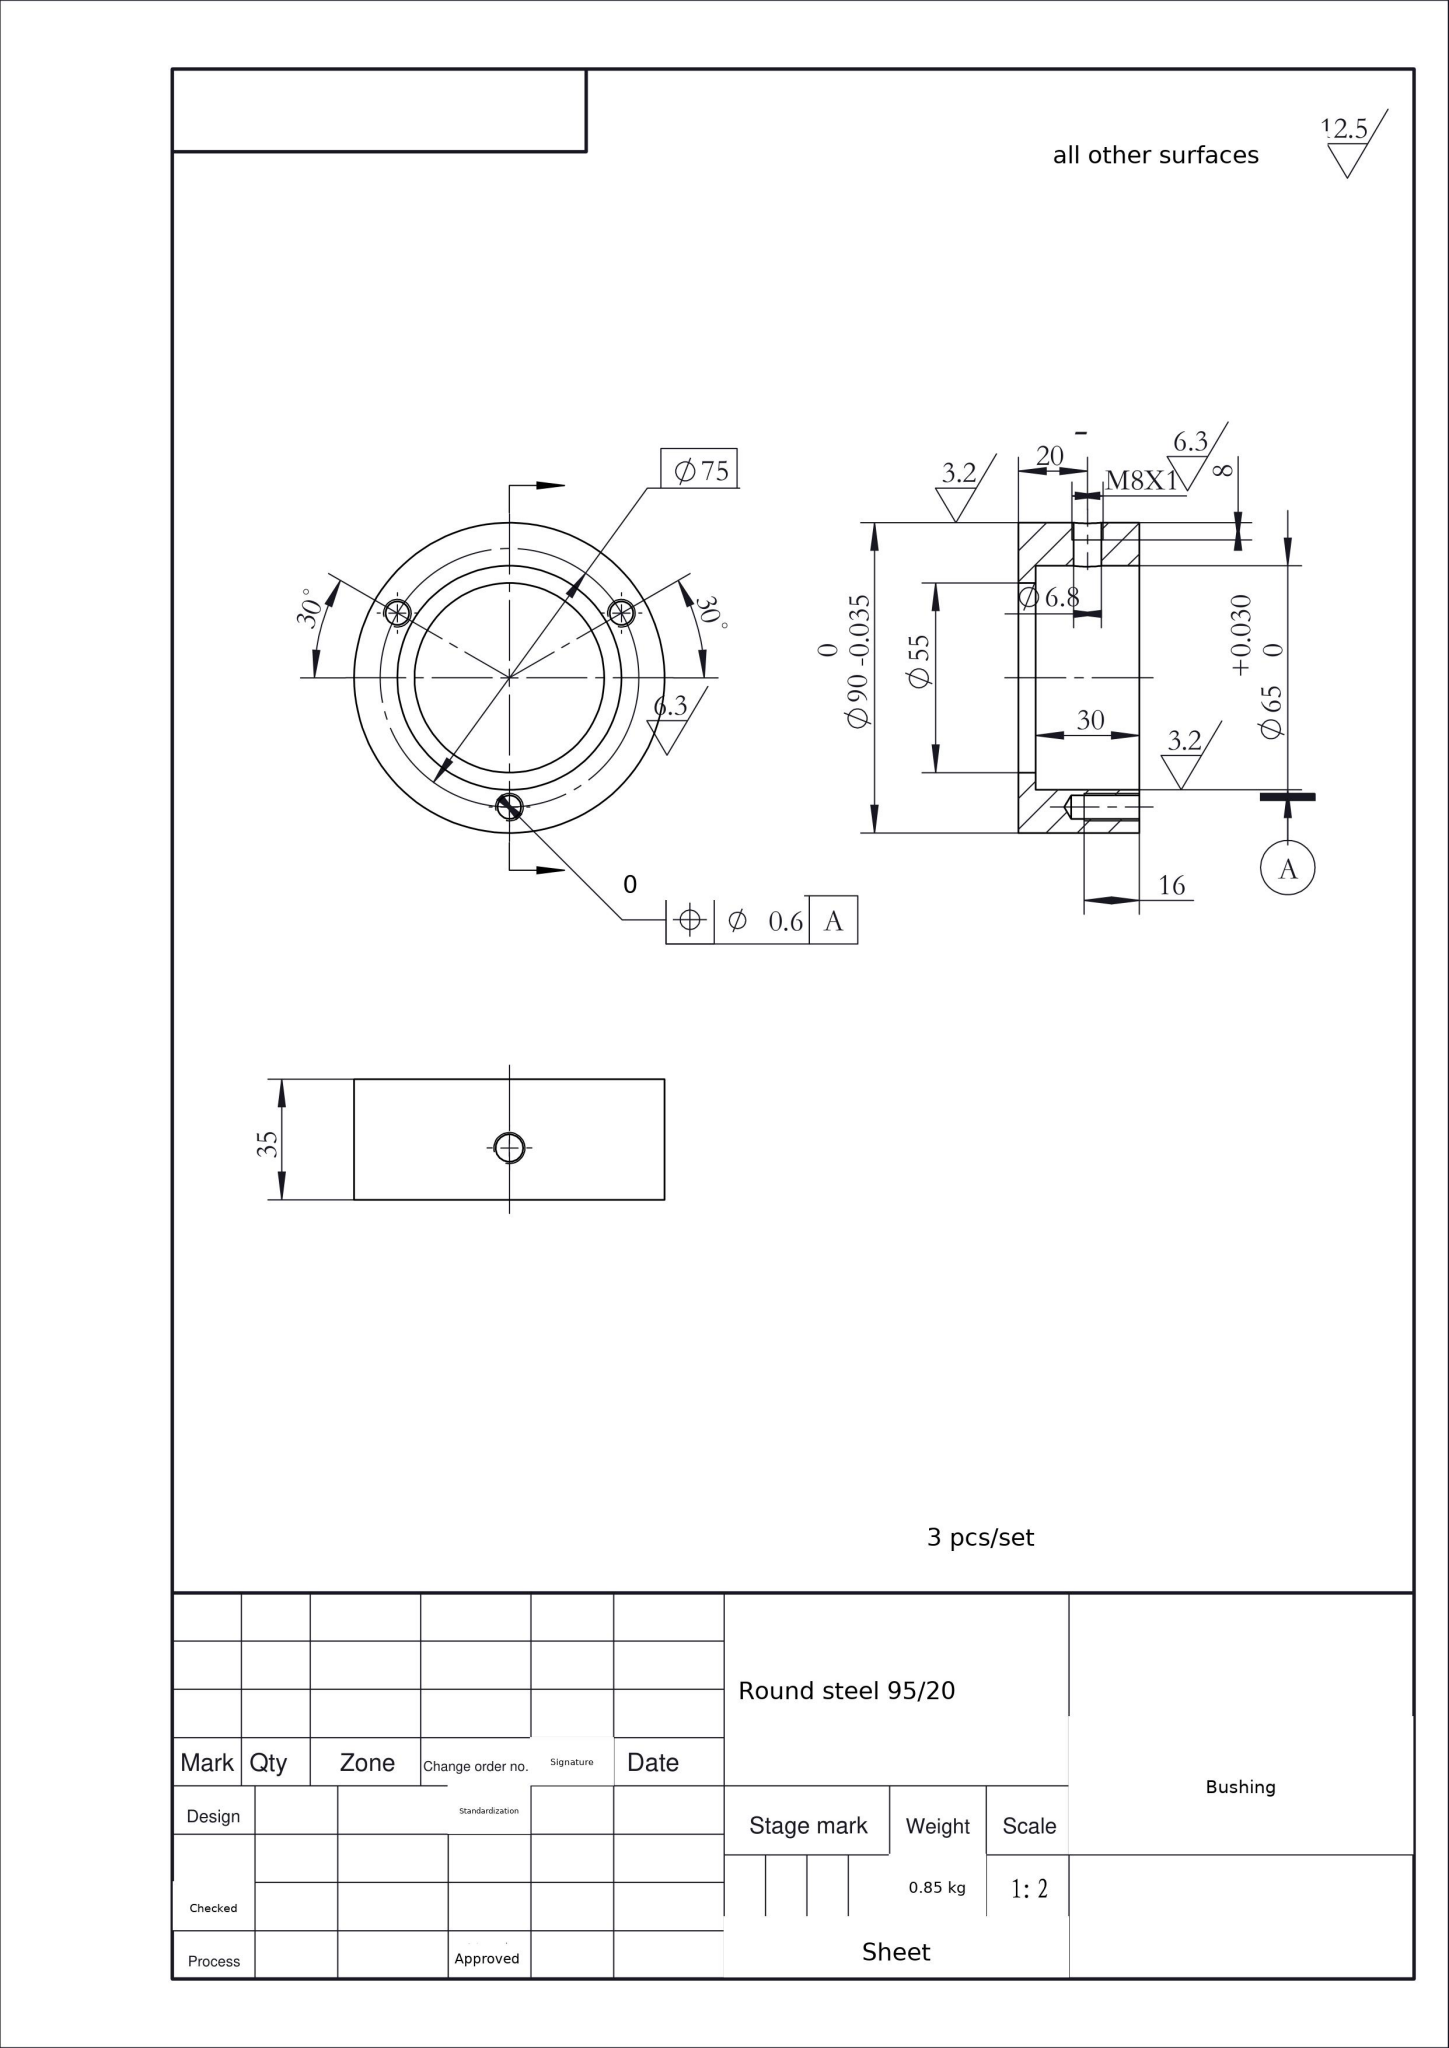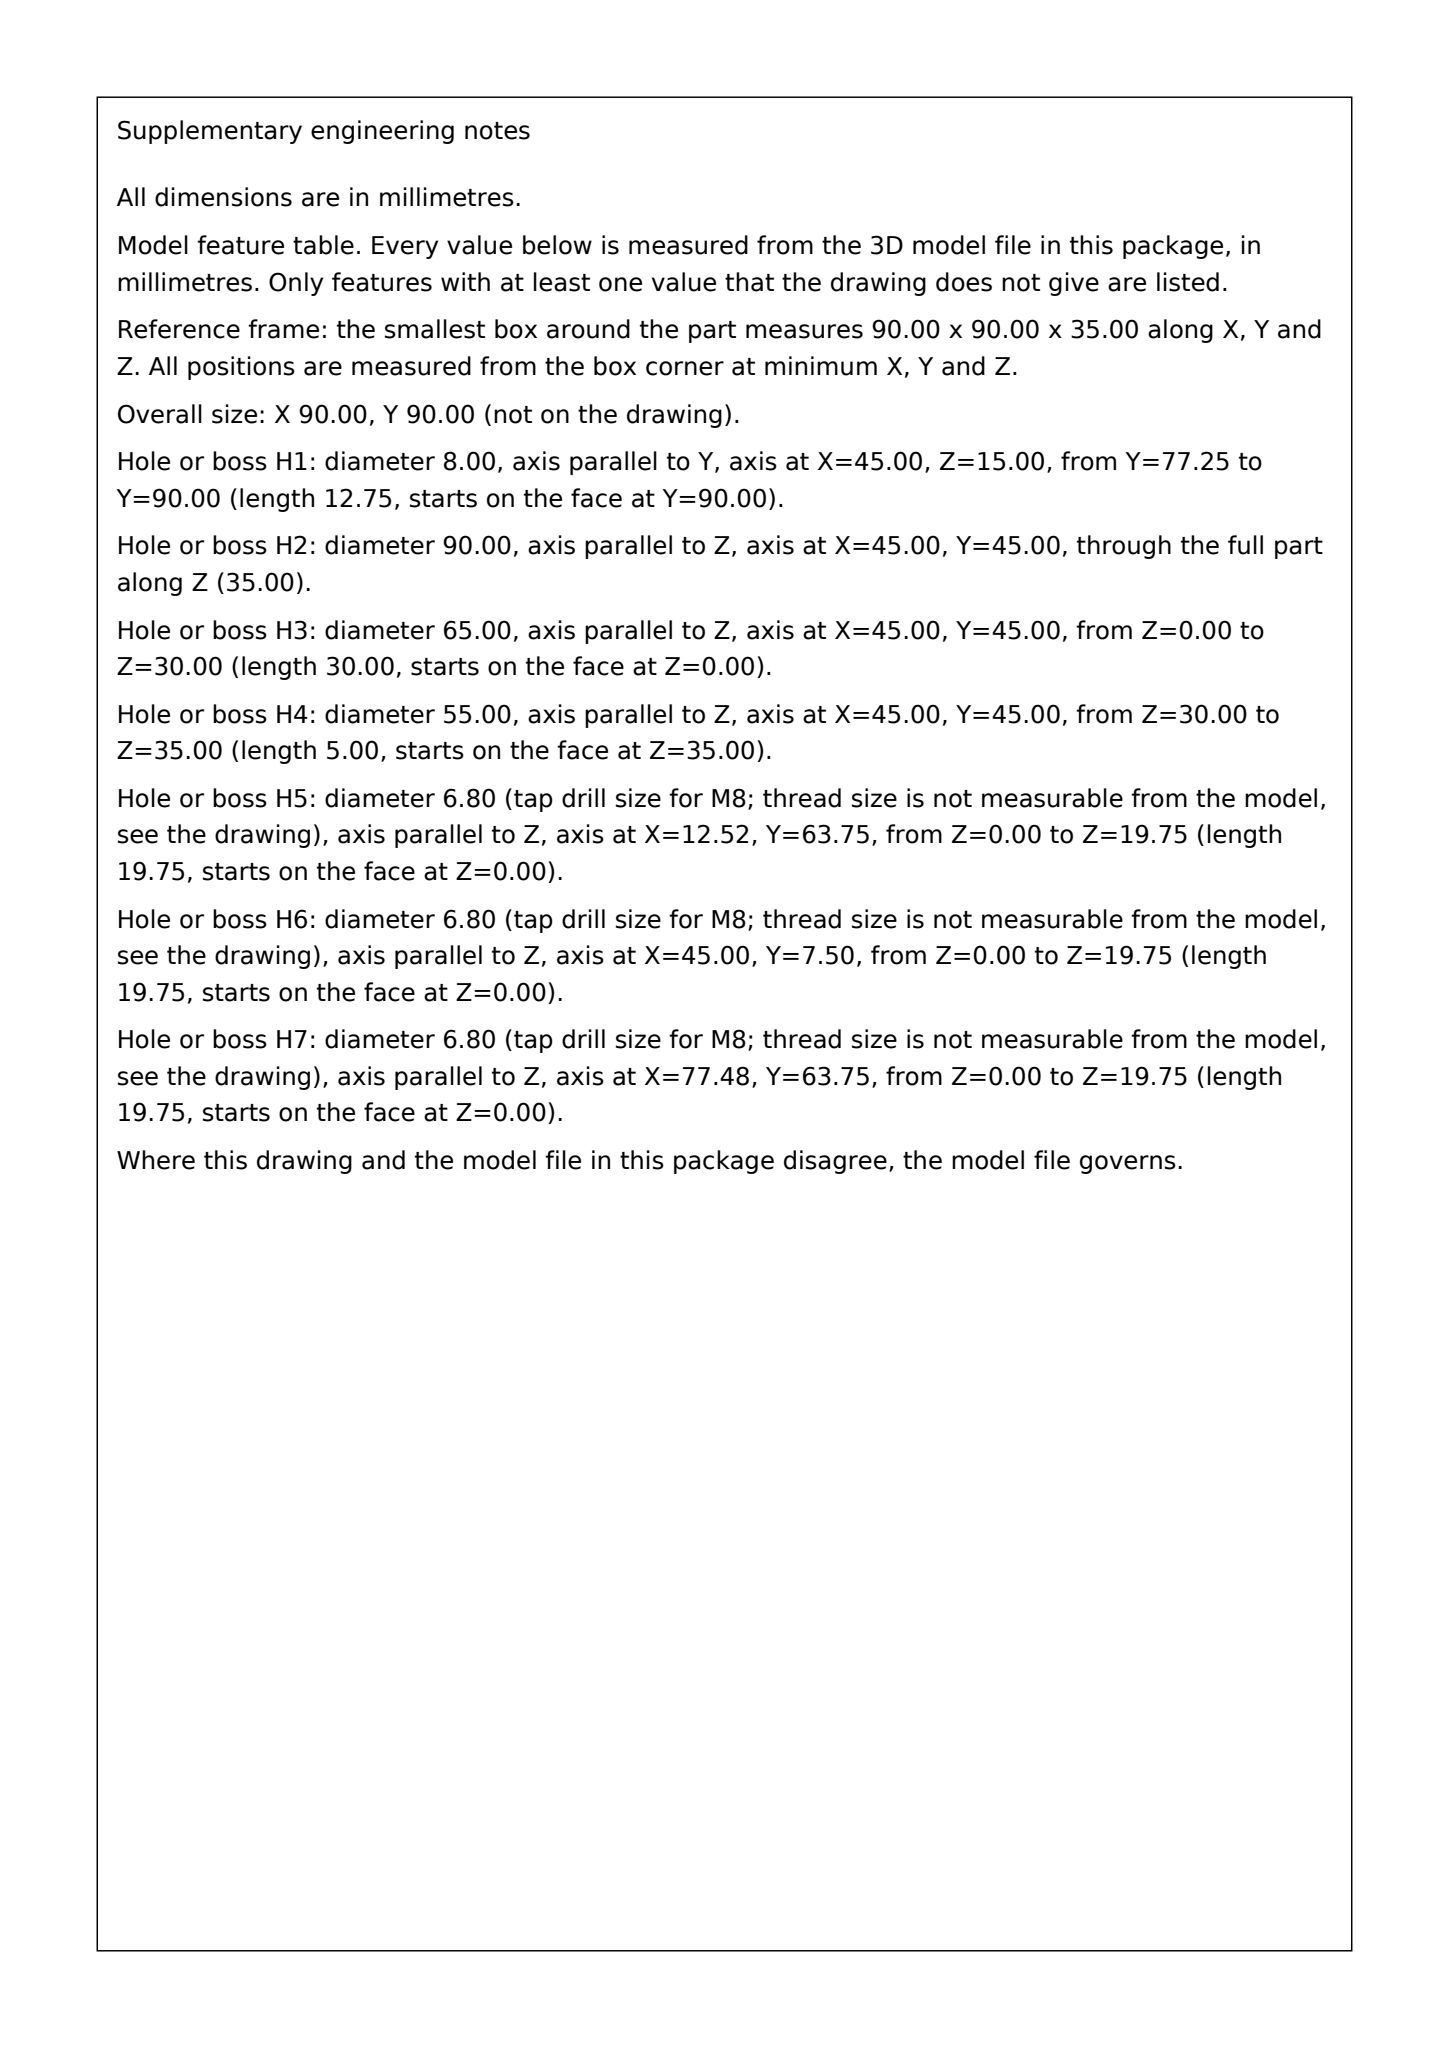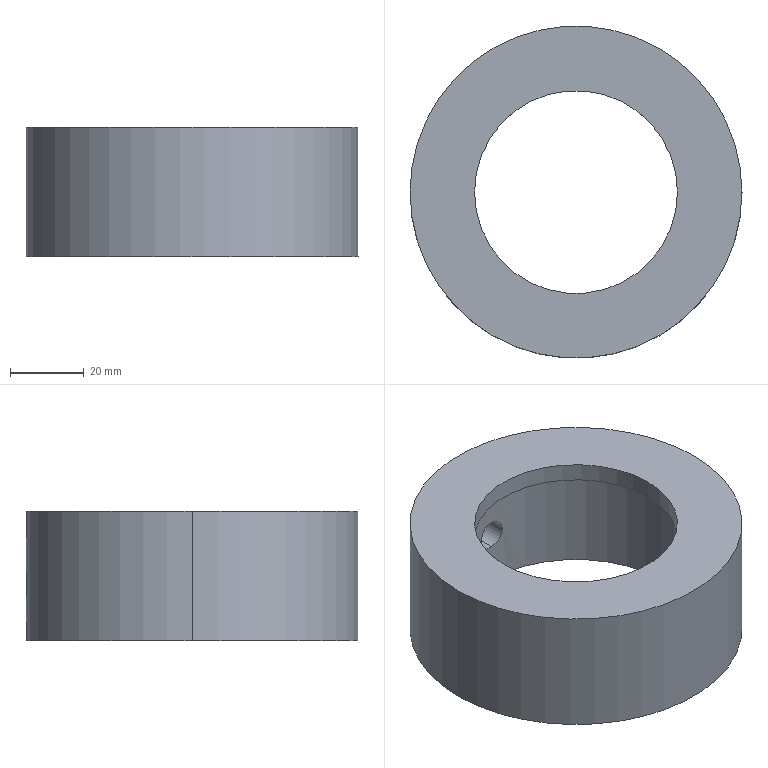Part | SolidWorks | mm | material Round steel 95/20 | 1 solid | 23 faces | box 90 x 90 x 35 mm | volume 108376 mm3 | cylinder 14 | cone 6 | plane 3 | commonest cylinder face diameters 6.8 x6 8 x2 65 x2 55 x2 90 x2
build123d program:
from build123d import *

# Parameters (mm, degrees)
SKETCH1_R               = 45
BOSS_EXTRUDE1_DEPTH     = 35
SKETCH2_R               = 27.5
CUT_EXTRUDE1_DEPTH      = 5
SKETCH3_R               = 32.5
CUT_EXTRUDE2_DEPTH      = 30
M8_TAPPED_HOLE1_D       = 6.8
M8_TAPPED_HOLE1_DEPTH   = 19.75
M8_TAPPED_HOLE1_TIP     = 2.043
CUT_EXTRUDE3_REACH      = 108.536
CUT_EXTRUDE3_END_RADIUS = 32.5
SKETCH9_R               = 4


with BuildPart() as part:
    # Sketch1 → Boss-Extrude1 (new body)
    with BuildSketch(Plane.XY):
        Circle(SKETCH1_R)
    extrude(amount=BOSS_EXTRUDE1_DEPTH)

    # Sketch2 → Cut-Extrude1 (cut)
    with BuildSketch(Plane.XY.offset(35)):
        Circle(SKETCH2_R)
    extrude(amount=-CUT_EXTRUDE1_DEPTH, mode=Mode.SUBTRACT)

    # Sketch3 → Cut-Extrude2 (cut)
    with BuildSketch(Plane(origin=(0, 0, 0), x_dir=(-1, 0, 0), z_dir=(0, 0, -1))):
        Circle(SKETCH3_R)
    extrude(amount=-CUT_EXTRUDE2_DEPTH, mode=Mode.SUBTRACT)

    # M8 Tapped Hole1
    with Locations(Plane(origin=(32.476, 18.75, 0), x_dir=(-1, 0, 0), z_dir=(0, 0, -1))):
        with Locations((0, 0), (64.952, 0), (32.476, -56.25)):
            Hole(M8_TAPPED_HOLE1_D / 2, depth=M8_TAPPED_HOLE1_DEPTH)
            with Locations((0, 0, -(M8_TAPPED_HOLE1_DEPTH + M8_TAPPED_HOLE1_TIP / 2))):  # 118° drill point
                Cone(0, M8_TAPPED_HOLE1_D / 2, M8_TAPPED_HOLE1_TIP, mode=Mode.SUBTRACT)

    # Cut-Extrude3: up to this cylinder (the profile starts outside it)
    cut_extrude3_end = Plane(origin=(0, 0, 15), z_dir=(0, 0, -1)) * Cylinder(CUT_EXTRUDE3_END_RADIUS, 283.072, mode=Mode.PRIVATE)
    # Sketch9 → Cut-Extrude3 (cut, up to the surface)
    with BuildSketch(Plane(origin=(0, 45, 0), x_dir=(1, 0, 0), z_dir=(0, 1, 0)), mode=Mode.PRIVATE) as cut_extrude3_sk1:
        with Locations(Location((0, -15, 0), (0, 0, 270))):
            Circle(SKETCH9_R)
    cut_extrude3_tool1 = extrude(cut_extrude3_sk1.sketch, amount=-CUT_EXTRUDE3_REACH, mode=Mode.PRIVATE) - cut_extrude3_end
    add(cut_extrude3_tool1.solids().sort_by_distance((0, 45, 15))[0], mode=Mode.SUBTRACT)


solid = part.part
STEP:
#1=CARTESIAN_POINT('',(0.,32.5,19.));
#2=VERTEX_POINT('',#1);
#3=CARTESIAN_POINT('',(-0.,32.5,11.));
#4=VERTEX_POINT('',#3);
#5=CARTESIAN_POINT('',(0.,32.5,19.));
#6=CARTESIAN_POINT('',(-0.2646,32.5,19.));
#7=CARTESIAN_POINT('',(-0.5246,32.497,18.974));
#8=CARTESIAN_POINT('',(-1.036,32.484,18.872));
#9=CARTESIAN_POINT('',(-1.29,32.475,18.795));
#10=CARTESIAN_POINT('',(-1.775,32.452,18.594));
#11=CARTESIAN_POINT('',(-2.004,32.439,18.471));
#12=CARTESIAN_POINT('',(-2.439,32.409,18.181));
#13=CARTESIAN_POINT('',(-2.645,32.393,18.012));
#14=CARTESIAN_POINT('',(-3.013,32.361,17.643));
#15=CARTESIAN_POINT('',(-3.179,32.345,17.442));
#16=CARTESIAN_POINT('',(-3.471,32.314,17.005));
#17=CARTESIAN_POINT('',(-3.595,32.301,16.773));
#18=CARTESIAN_POINT('',(-3.795,32.278,16.291));
#19=CARTESIAN_POINT('',(-3.872,32.269,16.039));
#20=CARTESIAN_POINT('',(-3.974,32.256,15.522));
#21=CARTESIAN_POINT('',(-4.,32.253,15.263));
#22=CARTESIAN_POINT('',(-4.,32.253,14.74));
#23=CARTESIAN_POINT('',(-3.974,32.256,14.475));
#24=CARTESIAN_POINT('',(-3.872,32.269,13.962));
#25=CARTESIAN_POINT('',(-3.796,32.278,13.712));
#26=CARTESIAN_POINT('',(-3.596,32.301,13.228));
#27=CARTESIAN_POINT('',(-3.47,32.315,12.994));
#28=CARTESIAN_POINT('',(-3.181,32.344,12.561));
#29=CARTESIAN_POINT('',(-3.015,32.36,12.359));
#30=CARTESIAN_POINT('',(-2.642,32.393,11.985));
#31=CARTESIAN_POINT('',(-2.44,32.409,11.82));
#32=CARTESIAN_POINT('',(-2.007,32.439,11.53));
#33=CARTESIAN_POINT('',(-1.773,32.452,11.405));
#34=CARTESIAN_POINT('',(-1.289,32.475,11.204));
#35=CARTESIAN_POINT('',(-1.04,32.484,11.129));
#36=CARTESIAN_POINT('',(-0.5265,32.497,11.026));
#37=CARTESIAN_POINT('',(-0.2612,32.5,11.));
#38=CARTESIAN_POINT('',(-0.,32.5,11.));
#39=B_SPLINE_CURVE_WITH_KNOTS('',3,(#5,#6,#7,#8,#9,#10,#11,#12,#13,#14,#15,#16,#17,#18,#19,#20,#21,#22,#23,#24,#25,#26,#27,#28,#29,#30,#31,#32,#33,#34,#35,#36,#37,#38),.UNSPECIFIED.,.F.,.F.,(4,2,2,2,2,2,2,2,2,2,2,2,2,2,2,2,4),(0.,0.0007824,0.001565,0.002347,0.003129,0.003912,0.004694,0.005476,0.006259,0.007041,0.007824,0.008606,0.009388,0.01017,0.01095,0.01174,0.01252),.UNSPECIFIED.);
#40=EDGE_CURVE('',#2,#4,#39,.T.);
#41=ORIENTED_EDGE('',*,*,#40,.T.);
#42=CARTESIAN_POINT('',(-0.,45.,11.));
#43=VERTEX_POINT('',#42);
#44=CARTESIAN_POINT('',(-0.,-45.001,11.));
#45=DIRECTION('',(-0.,1.,-0.));
#46=VECTOR('',#45,1000.);
#47=LINE('',#44,#46);
#48=EDGE_CURVE('',#4,#43,#47,.T.);
#49=ORIENTED_EDGE('',*,*,#48,.T.);
#50=CARTESIAN_POINT('',(-0.,45.,19.));
#51=VERTEX_POINT('',#50);
#52=CARTESIAN_POINT('',(-0.,45.,11.));
#53=CARTESIAN_POINT('',(-0.2611,45.,11.));
#54=CARTESIAN_POINT('',(-0.5206,44.998,11.025));
#55=CARTESIAN_POINT('',(-1.037,44.989,11.128));
#56=CARTESIAN_POINT('',(-1.289,44.982,11.205));
#57=CARTESIAN_POINT('',(-1.771,44.966,11.404));
#58=CARTESIAN_POINT('',(-2.003,44.956,11.528));
#59=CARTESIAN_POINT('',(-2.441,44.934,11.82));
#60=CARTESIAN_POINT('',(-2.642,44.923,11.985));
#61=CARTESIAN_POINT('',(-3.011,44.9,12.354));
#62=CARTESIAN_POINT('',(-3.18,44.888,12.559));
#63=CARTESIAN_POINT('',(-3.47,44.866,12.994));
#64=CARTESIAN_POINT('',(-3.593,44.856,13.224));
#65=CARTESIAN_POINT('',(-3.794,44.84,13.707));
#66=CARTESIAN_POINT('',(-3.872,44.833,13.962));
#67=CARTESIAN_POINT('',(-3.974,44.824,14.473));
#68=CARTESIAN_POINT('',(-4.,44.822,14.733));
#69=CARTESIAN_POINT('',(-4.,44.822,15.261));
#70=CARTESIAN_POINT('',(-3.974,44.824,15.522));
#71=CARTESIAN_POINT('',(-3.873,44.833,16.033));
#72=CARTESIAN_POINT('',(-3.796,44.84,16.287));
#73=CARTESIAN_POINT('',(-3.596,44.856,16.771));
#74=CARTESIAN_POINT('',(-3.473,44.866,17.001));
#75=CARTESIAN_POINT('',(-3.183,44.887,17.436));
#76=CARTESIAN_POINT('',(-3.015,44.899,17.642));
#77=CARTESIAN_POINT('',(-2.646,44.923,18.011));
#78=CARTESIAN_POINT('',(-2.445,44.934,18.177));
#79=CARTESIAN_POINT('',(-2.008,44.956,18.469));
#80=CARTESIAN_POINT('',(-1.776,44.966,18.594));
#81=CARTESIAN_POINT('',(-1.295,44.982,18.794));
#82=CARTESIAN_POINT('',(-1.043,44.989,18.871));
#83=CARTESIAN_POINT('',(-0.5259,44.998,18.974));
#84=CARTESIAN_POINT('',(-0.2644,45.,19.));
#85=CARTESIAN_POINT('',(-0.,45.,19.));
#86=B_SPLINE_CURVE_WITH_KNOTS('',3,(#52,#53,#54,#55,#56,#57,#58,#59,#60,#61,#62,#63,#64,#65,#66,#67,#68,#69,#70,#71,#72,#73,#74,#75,#76,#77,#78,#79,#80,#81,#82,#83,#84,#85),.UNSPECIFIED.,.F.,.F.,(4,2,2,2,2,2,2,2,2,2,2,2,2,2,2,2,4),(0.01251,0.01329,0.01408,0.01486,0.01564,0.01642,0.0172,0.01798,0.01877,0.01955,0.02033,0.02111,0.02189,0.02268,0.02346,0.02424,0.02502),.UNSPECIFIED.);
#87=EDGE_CURVE('',#43,#51,#86,.T.);
#88=ORIENTED_EDGE('',*,*,#87,.T.);
#89=CARTESIAN_POINT('',(-0.,-45.001,19.));
#90=DIRECTION('',(-0.,1.,-0.));
#91=VECTOR('',#90,1000.);
#92=LINE('',#89,#91);
#93=EDGE_CURVE('',#2,#51,#92,.T.);
#94=ORIENTED_EDGE('',*,*,#93,.F.);
#95=EDGE_LOOP('',(#41,#49,#88,#94));
#96=FACE_OUTER_BOUND('',#95,.T.);
#97=CARTESIAN_POINT('',(-0.,-45.001,15.));
#98=DIRECTION('',(-0.,1.,-0.));
#99=DIRECTION('',(-0.,0.,1.));
#100=AXIS2_PLACEMENT_3D('',#97,#98,#99);
#101=CYLINDRICAL_SURFACE('',#100,4.);
#102=ADVANCED_FACE('',(#96),#101,.F.);
#103=CARTESIAN_POINT('',(35.876,18.75,19.75));
#104=VERTEX_POINT('',#103);
#105=CARTESIAN_POINT('',(29.076,18.75,19.75));
#106=VERTEX_POINT('',#105);
#107=CARTESIAN_POINT('',(32.476,18.75,19.75));
#108=DIRECTION('',(0.,0.,-1.));
#109=DIRECTION('',(-1.,0.,0.));
#110=AXIS2_PLACEMENT_3D('',#107,#108,#109);
#111=CIRCLE('',#110,3.4);
#112=EDGE_CURVE('',#104,#106,#111,.T.);
#113=ORIENTED_EDGE('',*,*,#112,.F.);
#114=CARTESIAN_POINT('',(35.876,18.75,-0.));
#115=VERTEX_POINT('',#114);
#116=CARTESIAN_POINT('',(35.876,18.75,-0.));
#117=DIRECTION('',(0.,0.,-1.));
#118=VECTOR('',#117,1000.);
#119=LINE('',#116,#118);
#120=EDGE_CURVE('',#104,#115,#119,.T.);
#121=ORIENTED_EDGE('',*,*,#120,.T.);
#122=CARTESIAN_POINT('',(29.076,18.75,-0.));
#123=VERTEX_POINT('',#122);
#124=CARTESIAN_POINT('',(32.476,18.75,-0.));
#125=DIRECTION('',(0.,0.,-1.));
#126=DIRECTION('',(-1.,0.,0.));
#127=AXIS2_PLACEMENT_3D('',#124,#125,#126);
#128=CIRCLE('',#127,3.4);
#129=EDGE_CURVE('',#115,#123,#128,.T.);
#130=ORIENTED_EDGE('',*,*,#129,.T.);
#131=CARTESIAN_POINT('',(29.076,18.75,-0.));
#132=DIRECTION('',(0.,0.,-1.));
#133=VECTOR('',#132,1000.);
#134=LINE('',#131,#133);
#135=EDGE_CURVE('',#106,#123,#134,.T.);
#136=ORIENTED_EDGE('',*,*,#135,.F.);
#137=EDGE_LOOP('',(#113,#121,#130,#136));
#138=FACE_OUTER_BOUND('',#137,.T.);
#139=CARTESIAN_POINT('',(32.476,18.75,-0.));
#140=DIRECTION('',(0.,0.,-1.));
#141=DIRECTION('',(-1.,0.,0.));
#142=AXIS2_PLACEMENT_3D('',#139,#140,#141);
#143=CYLINDRICAL_SURFACE('',#142,3.4);
#144=ADVANCED_FACE('',(#138),#143,.F.);
#145=CARTESIAN_POINT('',(32.476,18.75,21.793));
#146=VERTEX_POINT('',#145);
#147=CARTESIAN_POINT('',(29.076,18.75,19.75));
#148=DIRECTION('',(-0.8572,0.,-0.515));
#149=VECTOR('',#148,1000.);
#150=LINE('',#147,#149);
#151=EDGE_CURVE('',#146,#106,#150,.T.);
#152=ORIENTED_EDGE('',*,*,#151,.F.);
#153=CARTESIAN_POINT('',(35.876,18.75,19.75));
#154=DIRECTION('',(0.8572,-0.,-0.515));
#155=VECTOR('',#154,1000.);
#156=LINE('',#153,#155);
#157=EDGE_CURVE('',#146,#104,#156,.T.);
#158=ORIENTED_EDGE('',*,*,#157,.T.);
#159=ORIENTED_EDGE('',*,*,#112,.T.);
#160=EDGE_LOOP('',(#152,#158,#159));
#161=FACE_OUTER_BOUND('',#160,.T.);
#162=CARTESIAN_POINT('',(32.476,18.75,19.75));
#163=DIRECTION('',(0.,0.,-1.));
#164=DIRECTION('',(-1.,0.,0.));
#165=AXIS2_PLACEMENT_3D('',#162,#163,#164);
#166=CONICAL_SURFACE('',#165,3.4,1.03);
#167=ADVANCED_FACE('',(#161),#166,.F.);
#168=CARTESIAN_POINT('',(-29.076,18.75,19.75));
#169=VERTEX_POINT('',#168);
#170=CARTESIAN_POINT('',(-35.876,18.75,19.75));
#171=VERTEX_POINT('',#170);
#172=CARTESIAN_POINT('',(-32.476,18.75,19.75));
#173=DIRECTION('',(0.,0.,-1.));
#174=DIRECTION('',(-1.,0.,0.));
#175=AXIS2_PLACEMENT_3D('',#172,#173,#174);
#176=CIRCLE('',#175,3.4);
#177=EDGE_CURVE('',#169,#171,#176,.T.);
#178=ORIENTED_EDGE('',*,*,#177,.F.);
#179=CARTESIAN_POINT('',(-29.076,18.75,-0.));
#180=VERTEX_POINT('',#179);
#181=CARTESIAN_POINT('',(-29.076,18.75,-0.));
#182=DIRECTION('',(0.,0.,-1.));
#183=VECTOR('',#182,1000.);
#184=LINE('',#181,#183);
#185=EDGE_CURVE('',#169,#180,#184,.T.);
#186=ORIENTED_EDGE('',*,*,#185,.T.);
#187=CARTESIAN_POINT('',(-35.876,18.75,-0.));
#188=VERTEX_POINT('',#187);
#189=CARTESIAN_POINT('',(-32.476,18.75,-0.));
#190=DIRECTION('',(0.,0.,-1.));
#191=DIRECTION('',(-1.,0.,0.));
#192=AXIS2_PLACEMENT_3D('',#189,#190,#191);
#193=CIRCLE('',#192,3.4);
#194=EDGE_CURVE('',#180,#188,#193,.T.);
#195=ORIENTED_EDGE('',*,*,#194,.T.);
#196=CARTESIAN_POINT('',(-35.876,18.75,-0.));
#197=DIRECTION('',(0.,0.,-1.));
#198=VECTOR('',#197,1000.);
#199=LINE('',#196,#198);
#200=EDGE_CURVE('',#171,#188,#199,.T.);
#201=ORIENTED_EDGE('',*,*,#200,.F.);
#202=EDGE_LOOP('',(#178,#186,#195,#201));
#203=FACE_OUTER_BOUND('',#202,.T.);
#204=CARTESIAN_POINT('',(-32.476,18.75,-0.));
#205=DIRECTION('',(0.,0.,-1.));
#206=DIRECTION('',(-1.,0.,0.));
#207=AXIS2_PLACEMENT_3D('',#204,#205,#206);
#208=CYLINDRICAL_SURFACE('',#207,3.4);
#209=ADVANCED_FACE('',(#203),#208,.F.);
#210=CARTESIAN_POINT('',(-32.476,18.75,21.793));
#211=VERTEX_POINT('',#210);
#212=CARTESIAN_POINT('',(-35.876,18.75,19.75));
#213=DIRECTION('',(-0.8572,0.,-0.515));
#214=VECTOR('',#213,1000.);
#215=LINE('',#212,#214);
#216=EDGE_CURVE('',#211,#171,#215,.T.);
#217=ORIENTED_EDGE('',*,*,#216,.F.);
#218=CARTESIAN_POINT('',(-29.076,18.75,19.75));
#219=DIRECTION('',(0.8572,-0.,-0.515));
#220=VECTOR('',#219,1000.);
#221=LINE('',#218,#220);
#222=EDGE_CURVE('',#211,#169,#221,.T.);
#223=ORIENTED_EDGE('',*,*,#222,.T.);
#224=ORIENTED_EDGE('',*,*,#177,.T.);
#225=EDGE_LOOP('',(#217,#223,#224));
#226=FACE_OUTER_BOUND('',#225,.T.);
#227=CARTESIAN_POINT('',(-32.476,18.75,19.75));
#228=DIRECTION('',(0.,0.,-1.));
#229=DIRECTION('',(-1.,0.,0.));
#230=AXIS2_PLACEMENT_3D('',#227,#228,#229);
#231=CONICAL_SURFACE('',#230,3.4,1.03);
#232=ADVANCED_FACE('',(#226),#231,.F.);
#233=CARTESIAN_POINT('',(3.4,-37.5,19.75));
#234=VERTEX_POINT('',#233);
#235=CARTESIAN_POINT('',(-3.4,-37.5,19.75));
#236=VERTEX_POINT('',#235);
#237=CARTESIAN_POINT('',(-0.,-37.5,19.75));
#238=DIRECTION('',(0.,0.,-1.));
#239=DIRECTION('',(-1.,0.,0.));
#240=AXIS2_PLACEMENT_3D('',#237,#238,#239);
#241=CIRCLE('',#240,3.4);
#242=EDGE_CURVE('',#234,#236,#241,.T.);
#243=ORIENTED_EDGE('',*,*,#242,.F.);
#244=CARTESIAN_POINT('',(3.4,-37.5,-0.));
#245=VERTEX_POINT('',#244);
#246=CARTESIAN_POINT('',(3.4,-37.5,-0.));
#247=DIRECTION('',(0.,0.,-1.));
#248=VECTOR('',#247,1000.);
#249=LINE('',#246,#248);
#250=EDGE_CURVE('',#234,#245,#249,.T.);
#251=ORIENTED_EDGE('',*,*,#250,.T.);
#252=CARTESIAN_POINT('',(-3.4,-37.5,-0.));
#253=VERTEX_POINT('',#252);
#254=CARTESIAN_POINT('',(-0.,-37.5,-0.));
#255=DIRECTION('',(0.,0.,-1.));
#256=DIRECTION('',(-1.,0.,0.));
#257=AXIS2_PLACEMENT_3D('',#254,#255,#256);
#258=CIRCLE('',#257,3.4);
#259=EDGE_CURVE('',#245,#253,#258,.T.);
#260=ORIENTED_EDGE('',*,*,#259,.T.);
#261=CARTESIAN_POINT('',(-3.4,-37.5,-0.));
#262=DIRECTION('',(0.,0.,-1.));
#263=VECTOR('',#262,1000.);
#264=LINE('',#261,#263);
#265=EDGE_CURVE('',#236,#253,#264,.T.);
#266=ORIENTED_EDGE('',*,*,#265,.F.);
#267=EDGE_LOOP('',(#243,#251,#260,#266));
#268=FACE_OUTER_BOUND('',#267,.T.);
#269=CARTESIAN_POINT('',(-0.,-37.5,-0.));
#270=DIRECTION('',(0.,0.,-1.));
#271=DIRECTION('',(-1.,0.,0.));
#272=AXIS2_PLACEMENT_3D('',#269,#270,#271);
#273=CYLINDRICAL_SURFACE('',#272,3.4);
#274=ADVANCED_FACE('',(#268),#273,.F.);
#275=CARTESIAN_POINT('',(-0.,-37.5,21.793));
#276=VERTEX_POINT('',#275);
#277=CARTESIAN_POINT('',(-3.4,-37.5,19.75));
#278=DIRECTION('',(-0.8572,0.,-0.515));
#279=VECTOR('',#278,1000.);
#280=LINE('',#277,#279);
#281=EDGE_CURVE('',#276,#236,#280,.T.);
#282=ORIENTED_EDGE('',*,*,#281,.F.);
#283=CARTESIAN_POINT('',(3.4,-37.5,19.75));
#284=DIRECTION('',(0.8572,-0.,-0.515));
#285=VECTOR('',#284,1000.);
#286=LINE('',#283,#285);
#287=EDGE_CURVE('',#276,#234,#286,.T.);
#288=ORIENTED_EDGE('',*,*,#287,.T.);
#289=ORIENTED_EDGE('',*,*,#242,.T.);
#290=EDGE_LOOP('',(#282,#288,#289));
#291=FACE_OUTER_BOUND('',#290,.T.);
#292=CARTESIAN_POINT('',(-0.,-37.5,19.75));
#293=DIRECTION('',(0.,0.,-1.));
#294=DIRECTION('',(-1.,0.,0.));
#295=AXIS2_PLACEMENT_3D('',#292,#293,#294);
#296=CONICAL_SURFACE('',#295,3.4,1.03);
#297=ADVANCED_FACE('',(#291),#296,.F.);
#298=CARTESIAN_POINT('',(32.5,-0.,30.));
#299=VERTEX_POINT('',#298);
#300=CARTESIAN_POINT('',(-32.5,-0.,30.));
#301=VERTEX_POINT('',#300);
#302=CARTESIAN_POINT('',(-0.,-0.,30.));
#303=DIRECTION('',(0.,0.,-1.));
#304=DIRECTION('',(-1.,0.,0.));
#305=AXIS2_PLACEMENT_3D('',#302,#303,#304);
#306=CIRCLE('',#305,32.5);
#307=EDGE_CURVE('',#299,#301,#306,.T.);
#308=ORIENTED_EDGE('',*,*,#307,.F.);
#309=CARTESIAN_POINT('',(32.5,-0.,0.));
#310=VERTEX_POINT('',#309);
#311=CARTESIAN_POINT('',(32.5,-0.,30.));
#312=DIRECTION('',(0.,0.,-1.));
#313=VECTOR('',#312,1000.);
#314=LINE('',#311,#313);
#315=EDGE_CURVE('',#299,#310,#314,.T.);
#316=ORIENTED_EDGE('',*,*,#315,.T.);
#317=CARTESIAN_POINT('',(-32.5,0.,0.));
#318=VERTEX_POINT('',#317);
#319=CARTESIAN_POINT('',(0.,0.,0.));
#320=DIRECTION('',(0.,0.,-1.));
#321=DIRECTION('',(-1.,0.,0.));
#322=AXIS2_PLACEMENT_3D('',#319,#320,#321);
#323=CIRCLE('',#322,32.5);
#324=EDGE_CURVE('',#310,#318,#323,.T.);
#325=ORIENTED_EDGE('',*,*,#324,.T.);
#326=CARTESIAN_POINT('',(-32.5,-0.,30.));
#327=DIRECTION('',(0.,0.,-1.));
#328=VECTOR('',#327,1000.);
#329=LINE('',#326,#328);
#330=EDGE_CURVE('',#301,#318,#329,.T.);
#331=ORIENTED_EDGE('',*,*,#330,.F.);
#332=EDGE_LOOP('',(#308,#316,#325,#331));
#333=FACE_OUTER_BOUND('',#332,.T.);
#334=CARTESIAN_POINT('',(-0.,-0.,30.));
#335=DIRECTION('',(0.,0.,-1.));
#336=DIRECTION('',(-1.,0.,0.));
#337=AXIS2_PLACEMENT_3D('',#334,#335,#336);
#338=CYLINDRICAL_SURFACE('',#337,32.5);
#339=ADVANCED_FACE('',(#333),#338,.F.);
#340=CARTESIAN_POINT('',(-27.5,-0.,30.));
#341=VERTEX_POINT('',#340);
#342=CARTESIAN_POINT('',(27.5,-0.,30.));
#343=VERTEX_POINT('',#342);
#344=CARTESIAN_POINT('',(-0.,-0.,30.));
#345=DIRECTION('',(-0.,-0.,1.));
#346=DIRECTION('',(1.,-0.,-0.));
#347=AXIS2_PLACEMENT_3D('',#344,#345,#346);
#348=CIRCLE('',#347,27.5);
#349=EDGE_CURVE('',#341,#343,#348,.T.);
#350=ORIENTED_EDGE('',*,*,#349,.F.);
#351=CARTESIAN_POINT('',(-27.5,-0.,35.));
#352=VERTEX_POINT('',#351);
#353=CARTESIAN_POINT('',(-27.5,-0.,30.));
#354=DIRECTION('',(-0.,-0.,1.));
#355=VECTOR('',#354,1000.);
#356=LINE('',#353,#355);
#357=EDGE_CURVE('',#341,#352,#356,.T.);
#358=ORIENTED_EDGE('',*,*,#357,.T.);
#359=CARTESIAN_POINT('',(27.5,-0.,35.));
#360=VERTEX_POINT('',#359);
#361=CARTESIAN_POINT('',(-0.,-0.,35.));
#362=DIRECTION('',(-0.,-0.,1.));
#363=DIRECTION('',(1.,-0.,-0.));
#364=AXIS2_PLACEMENT_3D('',#361,#362,#363);
#365=CIRCLE('',#364,27.5);
#366=EDGE_CURVE('',#352,#360,#365,.T.);
#367=ORIENTED_EDGE('',*,*,#366,.T.);
#368=CARTESIAN_POINT('',(27.5,-0.,30.));
#369=DIRECTION('',(-0.,-0.,1.));
#370=VECTOR('',#369,1000.);
#371=LINE('',#368,#370);
#372=EDGE_CURVE('',#343,#360,#371,.T.);
#373=ORIENTED_EDGE('',*,*,#372,.F.);
#374=EDGE_LOOP('',(#350,#358,#367,#373));
#375=FACE_OUTER_BOUND('',#374,.T.);
#376=CARTESIAN_POINT('',(-0.,-0.,30.));
#377=DIRECTION('',(-0.,-0.,1.));
#378=DIRECTION('',(1.,-0.,-0.));
#379=AXIS2_PLACEMENT_3D('',#376,#377,#378);
#380=CYLINDRICAL_SURFACE('',#379,27.5);
#381=ADVANCED_FACE('',(#375),#380,.F.);
#382=CARTESIAN_POINT('',(-0.,45.,19.));
#383=CARTESIAN_POINT('',(0.2644,45.,19.));
#384=CARTESIAN_POINT('',(0.5244,44.998,18.974));
#385=CARTESIAN_POINT('',(1.036,44.989,18.872));
#386=CARTESIAN_POINT('',(1.29,44.982,18.795));
#387=CARTESIAN_POINT('',(1.774,44.966,18.594));
#388=CARTESIAN_POINT('',(2.004,44.956,18.472));
#389=CARTESIAN_POINT('',(2.439,44.934,18.181));
#390=CARTESIAN_POINT('',(2.645,44.923,18.012));
#391=CARTESIAN_POINT('',(3.013,44.899,17.643));
#392=CARTESIAN_POINT('',(3.179,44.888,17.442));
#393=CARTESIAN_POINT('',(3.471,44.866,17.005));
#394=CARTESIAN_POINT('',(3.595,44.856,16.772));
#395=CARTESIAN_POINT('',(3.795,44.84,16.291));
#396=CARTESIAN_POINT('',(3.872,44.833,16.039));
#397=CARTESIAN_POINT('',(3.975,44.824,15.522));
#398=CARTESIAN_POINT('',(4.,44.822,15.262));
#399=CARTESIAN_POINT('',(4.,44.822,14.74));
#400=CARTESIAN_POINT('',(3.974,44.824,14.475));
#401=CARTESIAN_POINT('',(3.872,44.833,13.962));
#402=CARTESIAN_POINT('',(3.796,44.84,13.713));
#403=CARTESIAN_POINT('',(3.596,44.856,13.228));
#404=CARTESIAN_POINT('',(3.471,44.866,12.994));
#405=CARTESIAN_POINT('',(3.181,44.888,12.561));
#406=CARTESIAN_POINT('',(3.016,44.899,12.359));
#407=CARTESIAN_POINT('',(2.642,44.923,11.985));
#408=CARTESIAN_POINT('',(2.44,44.934,11.82));
#409=CARTESIAN_POINT('',(2.007,44.956,11.53));
#410=CARTESIAN_POINT('',(1.773,44.966,11.405));
#411=CARTESIAN_POINT('',(1.289,44.982,11.204));
#412=CARTESIAN_POINT('',(1.039,44.989,11.129));
#413=CARTESIAN_POINT('',(0.5264,44.998,11.026));
#414=CARTESIAN_POINT('',(0.2611,45.,11.));
#415=CARTESIAN_POINT('',(-0.,45.,11.));
#416=B_SPLINE_CURVE_WITH_KNOTS('',3,(#382,#383,#384,#385,#386,#387,#388,#389,#390,#391,#392,#393,#394,#395,#396,#397,#398,#399,#400,#401,#402,#403,#404,#405,#406,#407,#408,#409,#410,#411,#412,#413,#414,#415),.UNSPECIFIED.,.F.,.F.,(4,2,2,2,2,2,2,2,2,2,2,2,2,2,2,2,4),(0.,0.000782,0.001564,0.002346,0.003128,0.00391,0.004692,0.005474,0.006256,0.007038,0.00782,0.008602,0.009384,0.01017,0.01095,0.01173,0.01251),.UNSPECIFIED.);
#417=EDGE_CURVE('',#51,#43,#416,.T.);
#418=ORIENTED_EDGE('',*,*,#417,.F.);
#419=ORIENTED_EDGE('',*,*,#87,.F.);
#420=EDGE_LOOP('',(#418,#419));
#421=FACE_BOUND('',#420,.T.);
#422=CARTESIAN_POINT('',(45.,-0.,35.));
#423=VERTEX_POINT('',#422);
#424=CARTESIAN_POINT('',(-45.,-0.,35.));
#425=VERTEX_POINT('',#424);
#426=CARTESIAN_POINT('',(-0.,-0.,35.));
#427=DIRECTION('',(-0.,-0.,1.));
#428=DIRECTION('',(1.,-0.,-0.));
#429=AXIS2_PLACEMENT_3D('',#426,#427,#428);
#430=CIRCLE('',#429,45.);
#431=EDGE_CURVE('',#423,#425,#430,.T.);
#432=ORIENTED_EDGE('',*,*,#431,.F.);
#433=CARTESIAN_POINT('',(45.,-0.,0.));
#434=VERTEX_POINT('',#433);
#435=CARTESIAN_POINT('',(45.,-0.,35.));
#436=DIRECTION('',(0.,0.,-1.));
#437=VECTOR('',#436,1000.);
#438=LINE('',#435,#437);
#439=EDGE_CURVE('',#423,#434,#438,.T.);
#440=ORIENTED_EDGE('',*,*,#439,.T.);
#441=CARTESIAN_POINT('',(-45.,-0.,-0.));
#442=VERTEX_POINT('',#441);
#443=CARTESIAN_POINT('',(0.,0.,0.));
#444=DIRECTION('',(-0.,-0.,1.));
#445=DIRECTION('',(1.,-0.,-0.));
#446=AXIS2_PLACEMENT_3D('',#443,#444,#445);
#447=CIRCLE('',#446,45.);
#448=EDGE_CURVE('',#434,#442,#447,.T.);
#449=ORIENTED_EDGE('',*,*,#448,.T.);
#450=CARTESIAN_POINT('',(-45.,-0.,35.));
#451=DIRECTION('',(0.,0.,-1.));
#452=VECTOR('',#451,1000.);
#453=LINE('',#450,#452);
#454=EDGE_CURVE('',#425,#442,#453,.T.);
#455=ORIENTED_EDGE('',*,*,#454,.F.);
#456=EDGE_LOOP('',(#432,#440,#449,#455));
#457=FACE_OUTER_BOUND('',#456,.T.);
#458=CARTESIAN_POINT('',(-0.,-0.,35.));
#459=DIRECTION('',(0.,0.,-1.));
#460=DIRECTION('',(-1.,0.,0.));
#461=AXIS2_PLACEMENT_3D('',#458,#459,#460);
#462=CYLINDRICAL_SURFACE('',#461,45.);
#463=ADVANCED_FACE('',(#421,#457),#462,.T.);
#464=ORIENTED_EDGE('',*,*,#439,.F.);
#465=CARTESIAN_POINT('',(-0.,-0.,35.));
#466=DIRECTION('',(-0.,-0.,1.));
#467=DIRECTION('',(1.,-0.,-0.));
#468=AXIS2_PLACEMENT_3D('',#465,#466,#467);
#469=CIRCLE('',#468,45.);
#470=EDGE_CURVE('',#425,#423,#469,.T.);
#471=ORIENTED_EDGE('',*,*,#470,.F.);
#472=ORIENTED_EDGE('',*,*,#454,.T.);
#473=CARTESIAN_POINT('',(0.,0.,0.));
#474=DIRECTION('',(-0.,-0.,1.));
#475=DIRECTION('',(1.,-0.,-0.));
#476=AXIS2_PLACEMENT_3D('',#473,#474,#475);
#477=CIRCLE('',#476,45.);
#478=EDGE_CURVE('',#442,#434,#477,.T.);
#479=ORIENTED_EDGE('',*,*,#478,.T.);
#480=EDGE_LOOP('',(#464,#471,#472,#479));
#481=FACE_OUTER_BOUND('',#480,.T.);
#482=CARTESIAN_POINT('',(-0.,-0.,35.));
#483=DIRECTION('',(0.,0.,-1.));
#484=DIRECTION('',(-1.,0.,0.));
#485=AXIS2_PLACEMENT_3D('',#482,#483,#484);
#486=CYLINDRICAL_SURFACE('',#485,45.);
#487=ADVANCED_FACE('',(#481),#486,.T.);
#488=CARTESIAN_POINT('',(-0.,-0.,35.));
#489=DIRECTION('',(-0.,-0.,1.));
#490=DIRECTION('',(1.,-0.,-0.));
#491=AXIS2_PLACEMENT_3D('',#488,#489,#490);
#492=CIRCLE('',#491,27.5);
#493=EDGE_CURVE('',#360,#352,#492,.T.);
#494=ORIENTED_EDGE('',*,*,#493,.F.);
#495=ORIENTED_EDGE('',*,*,#366,.F.);
#496=EDGE_LOOP('',(#494,#495));
#497=FACE_BOUND('',#496,.T.);
#498=ORIENTED_EDGE('',*,*,#470,.T.);
#499=ORIENTED_EDGE('',*,*,#431,.T.);
#500=EDGE_LOOP('',(#498,#499));
#501=FACE_OUTER_BOUND('',#500,.T.);
#502=CARTESIAN_POINT('',(-0.,-0.,35.));
#503=DIRECTION('',(0.,-0.,1.));
#504=DIRECTION('',(1.,-0.,-0.));
#505=AXIS2_PLACEMENT_3D('',#502,#503,#504);
#506=PLANE('',#505);
#507=ADVANCED_FACE('',(#497,#501),#506,.T.);
#508=CARTESIAN_POINT('',(32.476,18.75,-0.));
#509=DIRECTION('',(0.,0.,-1.));
#510=DIRECTION('',(-1.,0.,0.));
#511=AXIS2_PLACEMENT_3D('',#508,#509,#510);
#512=CIRCLE('',#511,3.4);
#513=EDGE_CURVE('',#123,#115,#512,.T.);
#514=ORIENTED_EDGE('',*,*,#513,.F.);
#515=ORIENTED_EDGE('',*,*,#129,.F.);
#516=EDGE_LOOP('',(#514,#515));
#517=FACE_BOUND('',#516,.T.);
#518=CARTESIAN_POINT('',(-32.476,18.75,-0.));
#519=DIRECTION('',(0.,0.,-1.));
#520=DIRECTION('',(-1.,0.,0.));
#521=AXIS2_PLACEMENT_3D('',#518,#519,#520);
#522=CIRCLE('',#521,3.4);
#523=EDGE_CURVE('',#188,#180,#522,.T.);
#524=ORIENTED_EDGE('',*,*,#523,.F.);
#525=ORIENTED_EDGE('',*,*,#194,.F.);
#526=EDGE_LOOP('',(#524,#525));
#527=FACE_BOUND('',#526,.T.);
#528=CARTESIAN_POINT('',(-0.,-37.5,-0.));
#529=DIRECTION('',(0.,0.,-1.));
#530=DIRECTION('',(-1.,0.,0.));
#531=AXIS2_PLACEMENT_3D('',#528,#529,#530);
#532=CIRCLE('',#531,3.4);
#533=EDGE_CURVE('',#253,#245,#532,.T.);
#534=ORIENTED_EDGE('',*,*,#533,.F.);
#535=ORIENTED_EDGE('',*,*,#259,.F.);
#536=EDGE_LOOP('',(#534,#535));
#537=FACE_BOUND('',#536,.T.);
#538=CARTESIAN_POINT('',(0.,0.,0.));
#539=DIRECTION('',(0.,0.,-1.));
#540=DIRECTION('',(-1.,0.,0.));
#541=AXIS2_PLACEMENT_3D('',#538,#539,#540);
#542=CIRCLE('',#541,32.5);
#543=EDGE_CURVE('',#318,#310,#542,.T.);
#544=ORIENTED_EDGE('',*,*,#543,.F.);
#545=ORIENTED_EDGE('',*,*,#324,.F.);
#546=EDGE_LOOP('',(#544,#545));
#547=FACE_BOUND('',#546,.T.);
#548=ORIENTED_EDGE('',*,*,#478,.F.);
#549=ORIENTED_EDGE('',*,*,#448,.F.);
#550=EDGE_LOOP('',(#548,#549));
#551=FACE_OUTER_BOUND('',#550,.T.);
#552=CARTESIAN_POINT('',(0.,0.,0.));
#553=DIRECTION('',(0.,-0.,1.));
#554=DIRECTION('',(1.,-0.,-0.));
#555=AXIS2_PLACEMENT_3D('',#552,#553,#554);
#556=PLANE('',#555);
#557=ADVANCED_FACE('',(#517,#527,#537,#547,#551),#556,.F.);
#558=ORIENTED_EDGE('',*,*,#357,.F.);
#559=CARTESIAN_POINT('',(-0.,-0.,30.));
#560=DIRECTION('',(-0.,-0.,1.));
#561=DIRECTION('',(1.,-0.,-0.));
#562=AXIS2_PLACEMENT_3D('',#559,#560,#561);
#563=CIRCLE('',#562,27.5);
#564=EDGE_CURVE('',#343,#341,#563,.T.);
#565=ORIENTED_EDGE('',*,*,#564,.F.);
#566=ORIENTED_EDGE('',*,*,#372,.T.);
#567=ORIENTED_EDGE('',*,*,#493,.T.);
#568=EDGE_LOOP('',(#558,#565,#566,#567));
#569=FACE_OUTER_BOUND('',#568,.T.);
#570=CARTESIAN_POINT('',(-0.,-0.,30.));
#571=DIRECTION('',(-0.,-0.,1.));
#572=DIRECTION('',(1.,-0.,-0.));
#573=AXIS2_PLACEMENT_3D('',#570,#571,#572);
#574=CYLINDRICAL_SURFACE('',#573,27.5);
#575=ADVANCED_FACE('',(#569),#574,.F.);
#576=CARTESIAN_POINT('',(-0.,-0.,30.));
#577=DIRECTION('',(0.,0.,-1.));
#578=DIRECTION('',(-1.,0.,0.));
#579=AXIS2_PLACEMENT_3D('',#576,#577,#578);
#580=CIRCLE('',#579,32.5);
#581=EDGE_CURVE('',#301,#299,#580,.T.);
#582=ORIENTED_EDGE('',*,*,#581,.T.);
#583=ORIENTED_EDGE('',*,*,#307,.T.);
#584=EDGE_LOOP('',(#582,#583));
#585=FACE_OUTER_BOUND('',#584,.T.);
#586=ORIENTED_EDGE('',*,*,#564,.T.);
#587=ORIENTED_EDGE('',*,*,#349,.T.);
#588=EDGE_LOOP('',(#586,#587));
#589=FACE_BOUND('',#588,.T.);
#590=CARTESIAN_POINT('',(-0.,-0.,30.));
#591=DIRECTION('',(-0.,0.,-1.));
#592=DIRECTION('',(-1.,0.,0.));
#593=AXIS2_PLACEMENT_3D('',#590,#591,#592);
#594=PLANE('',#593);
#595=ADVANCED_FACE('',(#585,#589),#594,.T.);
#596=ORIENTED_EDGE('',*,*,#315,.F.);
#597=ORIENTED_EDGE('',*,*,#581,.F.);
#598=ORIENTED_EDGE('',*,*,#330,.T.);
#599=ORIENTED_EDGE('',*,*,#543,.T.);
#600=EDGE_LOOP('',(#596,#597,#598,#599));
#601=FACE_OUTER_BOUND('',#600,.T.);
#602=ORIENTED_EDGE('',*,*,#40,.F.);
#603=CARTESIAN_POINT('',(-0.,32.5,11.));
#604=CARTESIAN_POINT('',(0.2611,32.5,11.));
#605=CARTESIAN_POINT('',(0.5208,32.497,11.025));
#606=CARTESIAN_POINT('',(1.037,32.484,11.128));
#607=CARTESIAN_POINT('',(1.29,32.475,11.205));
#608=CARTESIAN_POINT('',(1.771,32.453,11.404));
#609=CARTESIAN_POINT('',(2.004,32.439,11.528));
#610=CARTESIAN_POINT('',(2.441,32.409,11.82));
#611=CARTESIAN_POINT('',(2.642,32.393,11.985));
#612=CARTESIAN_POINT('',(3.011,32.361,12.354));
#613=CARTESIAN_POINT('',(3.18,32.344,12.559));
#614=CARTESIAN_POINT('',(3.47,32.315,12.994));
#615=CARTESIAN_POINT('',(3.593,32.301,13.223));
#616=CARTESIAN_POINT('',(3.794,32.278,13.707));
#617=CARTESIAN_POINT('',(3.872,32.269,13.961));
#618=CARTESIAN_POINT('',(3.974,32.256,14.473));
#619=CARTESIAN_POINT('',(4.,32.253,14.733));
#620=CARTESIAN_POINT('',(4.,32.253,15.262));
#621=CARTESIAN_POINT('',(3.974,32.256,15.522));
#622=CARTESIAN_POINT('',(3.873,32.268,16.033));
#623=CARTESIAN_POINT('',(3.796,32.278,16.287));
#624=CARTESIAN_POINT('',(3.596,32.301,16.772));
#625=CARTESIAN_POINT('',(3.473,32.314,17.002));
#626=CARTESIAN_POINT('',(3.183,32.344,17.436));
#627=CARTESIAN_POINT('',(3.015,32.36,17.642));
#628=CARTESIAN_POINT('',(2.646,32.393,18.011));
#629=CARTESIAN_POINT('',(2.445,32.409,18.177));
#630=CARTESIAN_POINT('',(2.008,32.439,18.469));
#631=CARTESIAN_POINT('',(1.776,32.452,18.594));
#632=CARTESIAN_POINT('',(1.295,32.475,18.794));
#633=CARTESIAN_POINT('',(1.043,32.484,18.871));
#634=CARTESIAN_POINT('',(0.526,32.497,18.974));
#635=CARTESIAN_POINT('',(0.2645,32.5,19.));
#636=CARTESIAN_POINT('',(0.,32.5,19.));
#637=B_SPLINE_CURVE_WITH_KNOTS('',3,(#603,#604,#605,#606,#607,#608,#609,#610,#611,#612,#613,#614,#615,#616,#617,#618,#619,#620,#621,#622,#623,#624,#625,#626,#627,#628,#629,#630,#631,#632,#633,#634,#635,#636),.UNSPECIFIED.,.F.,.F.,(4,2,2,2,2,2,2,2,2,2,2,2,2,2,2,2,4),(0.01252,0.0133,0.01408,0.01486,0.01565,0.01643,0.01721,0.01799,0.01878,0.01956,0.02034,0.02112,0.0219,0.02269,0.02347,0.02425,0.02503),.UNSPECIFIED.);
#638=EDGE_CURVE('',#4,#2,#637,.T.);
#639=ORIENTED_EDGE('',*,*,#638,.F.);
#640=EDGE_LOOP('',(#602,#639));
#641=FACE_BOUND('',#640,.T.);
#642=CARTESIAN_POINT('',(-0.,-0.,30.));
#643=DIRECTION('',(0.,0.,-1.));
#644=DIRECTION('',(-1.,0.,0.));
#645=AXIS2_PLACEMENT_3D('',#642,#643,#644);
#646=CYLINDRICAL_SURFACE('',#645,32.5);
#647=ADVANCED_FACE('',(#601,#641),#646,.F.);
#648=ORIENTED_EDGE('',*,*,#287,.F.);
#649=ORIENTED_EDGE('',*,*,#281,.T.);
#650=CARTESIAN_POINT('',(-0.,-37.5,19.75));
#651=DIRECTION('',(0.,0.,-1.));
#652=DIRECTION('',(-1.,0.,0.));
#653=AXIS2_PLACEMENT_3D('',#650,#651,#652);
#654=CIRCLE('',#653,3.4);
#655=EDGE_CURVE('',#236,#234,#654,.T.);
#656=ORIENTED_EDGE('',*,*,#655,.T.);
#657=EDGE_LOOP('',(#648,#649,#656));
#658=FACE_OUTER_BOUND('',#657,.T.);
#659=CARTESIAN_POINT('',(-0.,-37.5,19.75));
#660=DIRECTION('',(0.,0.,-1.));
#661=DIRECTION('',(-1.,0.,0.));
#662=AXIS2_PLACEMENT_3D('',#659,#660,#661);
#663=CONICAL_SURFACE('',#662,3.4,1.03);
#664=ADVANCED_FACE('',(#658),#663,.F.);
#665=ORIENTED_EDGE('',*,*,#250,.F.);
#666=ORIENTED_EDGE('',*,*,#655,.F.);
#667=ORIENTED_EDGE('',*,*,#265,.T.);
#668=ORIENTED_EDGE('',*,*,#533,.T.);
#669=EDGE_LOOP('',(#665,#666,#667,#668));
#670=FACE_OUTER_BOUND('',#669,.T.);
#671=CARTESIAN_POINT('',(-0.,-37.5,-0.));
#672=DIRECTION('',(0.,0.,-1.));
#673=DIRECTION('',(-1.,0.,0.));
#674=AXIS2_PLACEMENT_3D('',#671,#672,#673);
#675=CYLINDRICAL_SURFACE('',#674,3.4);
#676=ADVANCED_FACE('',(#670),#675,.F.);
#677=ORIENTED_EDGE('',*,*,#222,.F.);
#678=ORIENTED_EDGE('',*,*,#216,.T.);
#679=CARTESIAN_POINT('',(-32.476,18.75,19.75));
#680=DIRECTION('',(0.,0.,-1.));
#681=DIRECTION('',(-1.,0.,0.));
#682=AXIS2_PLACEMENT_3D('',#679,#680,#681);
#683=CIRCLE('',#682,3.4);
#684=EDGE_CURVE('',#171,#169,#683,.T.);
#685=ORIENTED_EDGE('',*,*,#684,.T.);
#686=EDGE_LOOP('',(#677,#678,#685));
#687=FACE_OUTER_BOUND('',#686,.T.);
#688=CARTESIAN_POINT('',(-32.476,18.75,19.75));
#689=DIRECTION('',(0.,0.,-1.));
#690=DIRECTION('',(-1.,0.,0.));
#691=AXIS2_PLACEMENT_3D('',#688,#689,#690);
#692=CONICAL_SURFACE('',#691,3.4,1.03);
#693=ADVANCED_FACE('',(#687),#692,.F.);
#694=ORIENTED_EDGE('',*,*,#185,.F.);
#695=ORIENTED_EDGE('',*,*,#684,.F.);
#696=ORIENTED_EDGE('',*,*,#200,.T.);
#697=ORIENTED_EDGE('',*,*,#523,.T.);
#698=EDGE_LOOP('',(#694,#695,#696,#697));
#699=FACE_OUTER_BOUND('',#698,.T.);
#700=CARTESIAN_POINT('',(-32.476,18.75,-0.));
#701=DIRECTION('',(0.,0.,-1.));
#702=DIRECTION('',(-1.,0.,0.));
#703=AXIS2_PLACEMENT_3D('',#700,#701,#702);
#704=CYLINDRICAL_SURFACE('',#703,3.4);
#705=ADVANCED_FACE('',(#699),#704,.F.);
#706=ORIENTED_EDGE('',*,*,#157,.F.);
#707=ORIENTED_EDGE('',*,*,#151,.T.);
#708=CARTESIAN_POINT('',(32.476,18.75,19.75));
#709=DIRECTION('',(0.,0.,-1.));
#710=DIRECTION('',(-1.,0.,0.));
#711=AXIS2_PLACEMENT_3D('',#708,#709,#710);
#712=CIRCLE('',#711,3.4);
#713=EDGE_CURVE('',#106,#104,#712,.T.);
#714=ORIENTED_EDGE('',*,*,#713,.T.);
#715=EDGE_LOOP('',(#706,#707,#714));
#716=FACE_OUTER_BOUND('',#715,.T.);
#717=CARTESIAN_POINT('',(32.476,18.75,19.75));
#718=DIRECTION('',(0.,0.,-1.));
#719=DIRECTION('',(-1.,0.,0.));
#720=AXIS2_PLACEMENT_3D('',#717,#718,#719);
#721=CONICAL_SURFACE('',#720,3.4,1.03);
#722=ADVANCED_FACE('',(#716),#721,.F.);
#723=ORIENTED_EDGE('',*,*,#120,.F.);
#724=ORIENTED_EDGE('',*,*,#713,.F.);
#725=ORIENTED_EDGE('',*,*,#135,.T.);
#726=ORIENTED_EDGE('',*,*,#513,.T.);
#727=EDGE_LOOP('',(#723,#724,#725,#726));
#728=FACE_OUTER_BOUND('',#727,.T.);
#729=CARTESIAN_POINT('',(32.476,18.75,-0.));
#730=DIRECTION('',(0.,0.,-1.));
#731=DIRECTION('',(-1.,0.,0.));
#732=AXIS2_PLACEMENT_3D('',#729,#730,#731);
#733=CYLINDRICAL_SURFACE('',#732,3.4);
#734=ADVANCED_FACE('',(#728),#733,.F.);
#735=ORIENTED_EDGE('',*,*,#48,.F.);
#736=ORIENTED_EDGE('',*,*,#638,.T.);
#737=ORIENTED_EDGE('',*,*,#93,.T.);
#738=ORIENTED_EDGE('',*,*,#417,.T.);
#739=EDGE_LOOP('',(#735,#736,#737,#738));
#740=FACE_OUTER_BOUND('',#739,.T.);
#741=CARTESIAN_POINT('',(-0.,-45.001,15.));
#742=DIRECTION('',(-0.,1.,-0.));
#743=DIRECTION('',(-0.,0.,1.));
#744=AXIS2_PLACEMENT_3D('',#741,#742,#743);
#745=CYLINDRICAL_SURFACE('',#744,4.);
#746=ADVANCED_FACE('',(#740),#745,.F.);
#747=CLOSED_SHELL('',(#102,#144,#167,#209,#232,#274,#297,#339,#381,#463,#487,#507,#557,#575,#595,#647,#664,#676,#693,#705,#722,#734,#746));
#748=MANIFOLD_SOLID_BREP('',#747);
#749=CARTESIAN_POINT('',(0.,0.,0.));
#750=DIRECTION('',(0.,0.,1.));
#751=DIRECTION('',(1.,0.,0.));
#752=AXIS2_PLACEMENT_3D('',#749,#750,#751);
#753=(LENGTH_UNIT()NAMED_UNIT(*)SI_UNIT(.MILLI.,.METRE.));
#754=UNCERTAINTY_MEASURE_WITH_UNIT(LENGTH_MEASURE(0.00001),#753,'','');
#755=(NAMED_UNIT(*)PLANE_ANGLE_UNIT()SI_UNIT($,.RADIAN.));
#756=(NAMED_UNIT(*)SI_UNIT($,.STERADIAN.)SOLID_ANGLE_UNIT());
#757=(GEOMETRIC_REPRESENTATION_CONTEXT(3)GLOBAL_UNCERTAINTY_ASSIGNED_CONTEXT((#754))GLOBAL_UNIT_ASSIGNED_CONTEXT((#753,#755,#756))REPRESENTATION_CONTEXT('',''));
#758=ADVANCED_BREP_SHAPE_REPRESENTATION('',(#748,#752),#757);